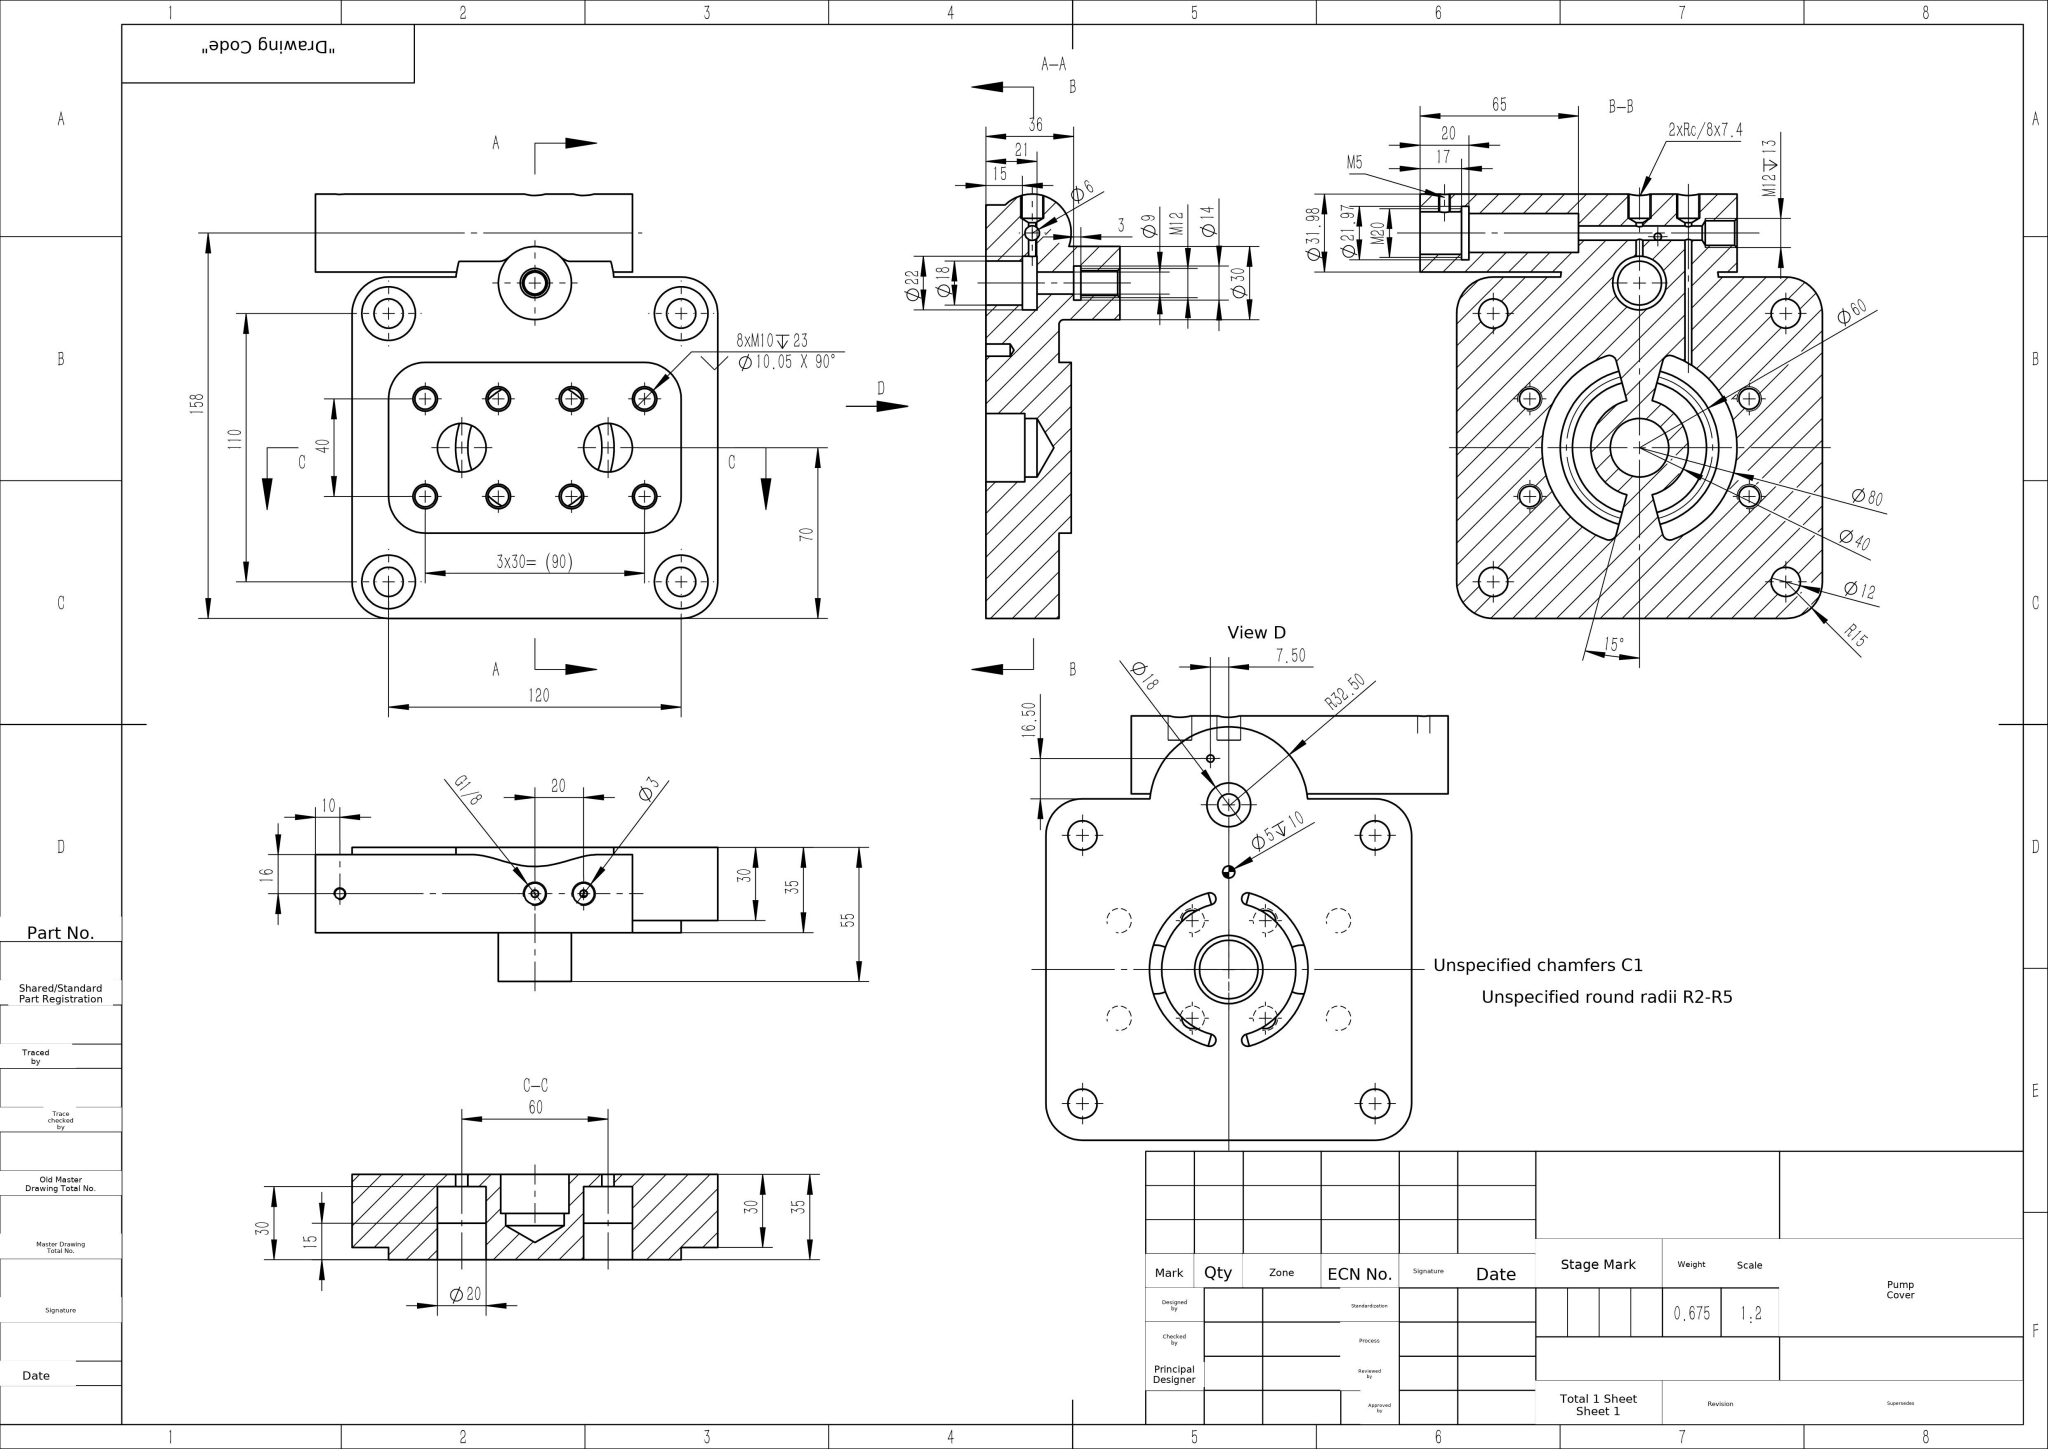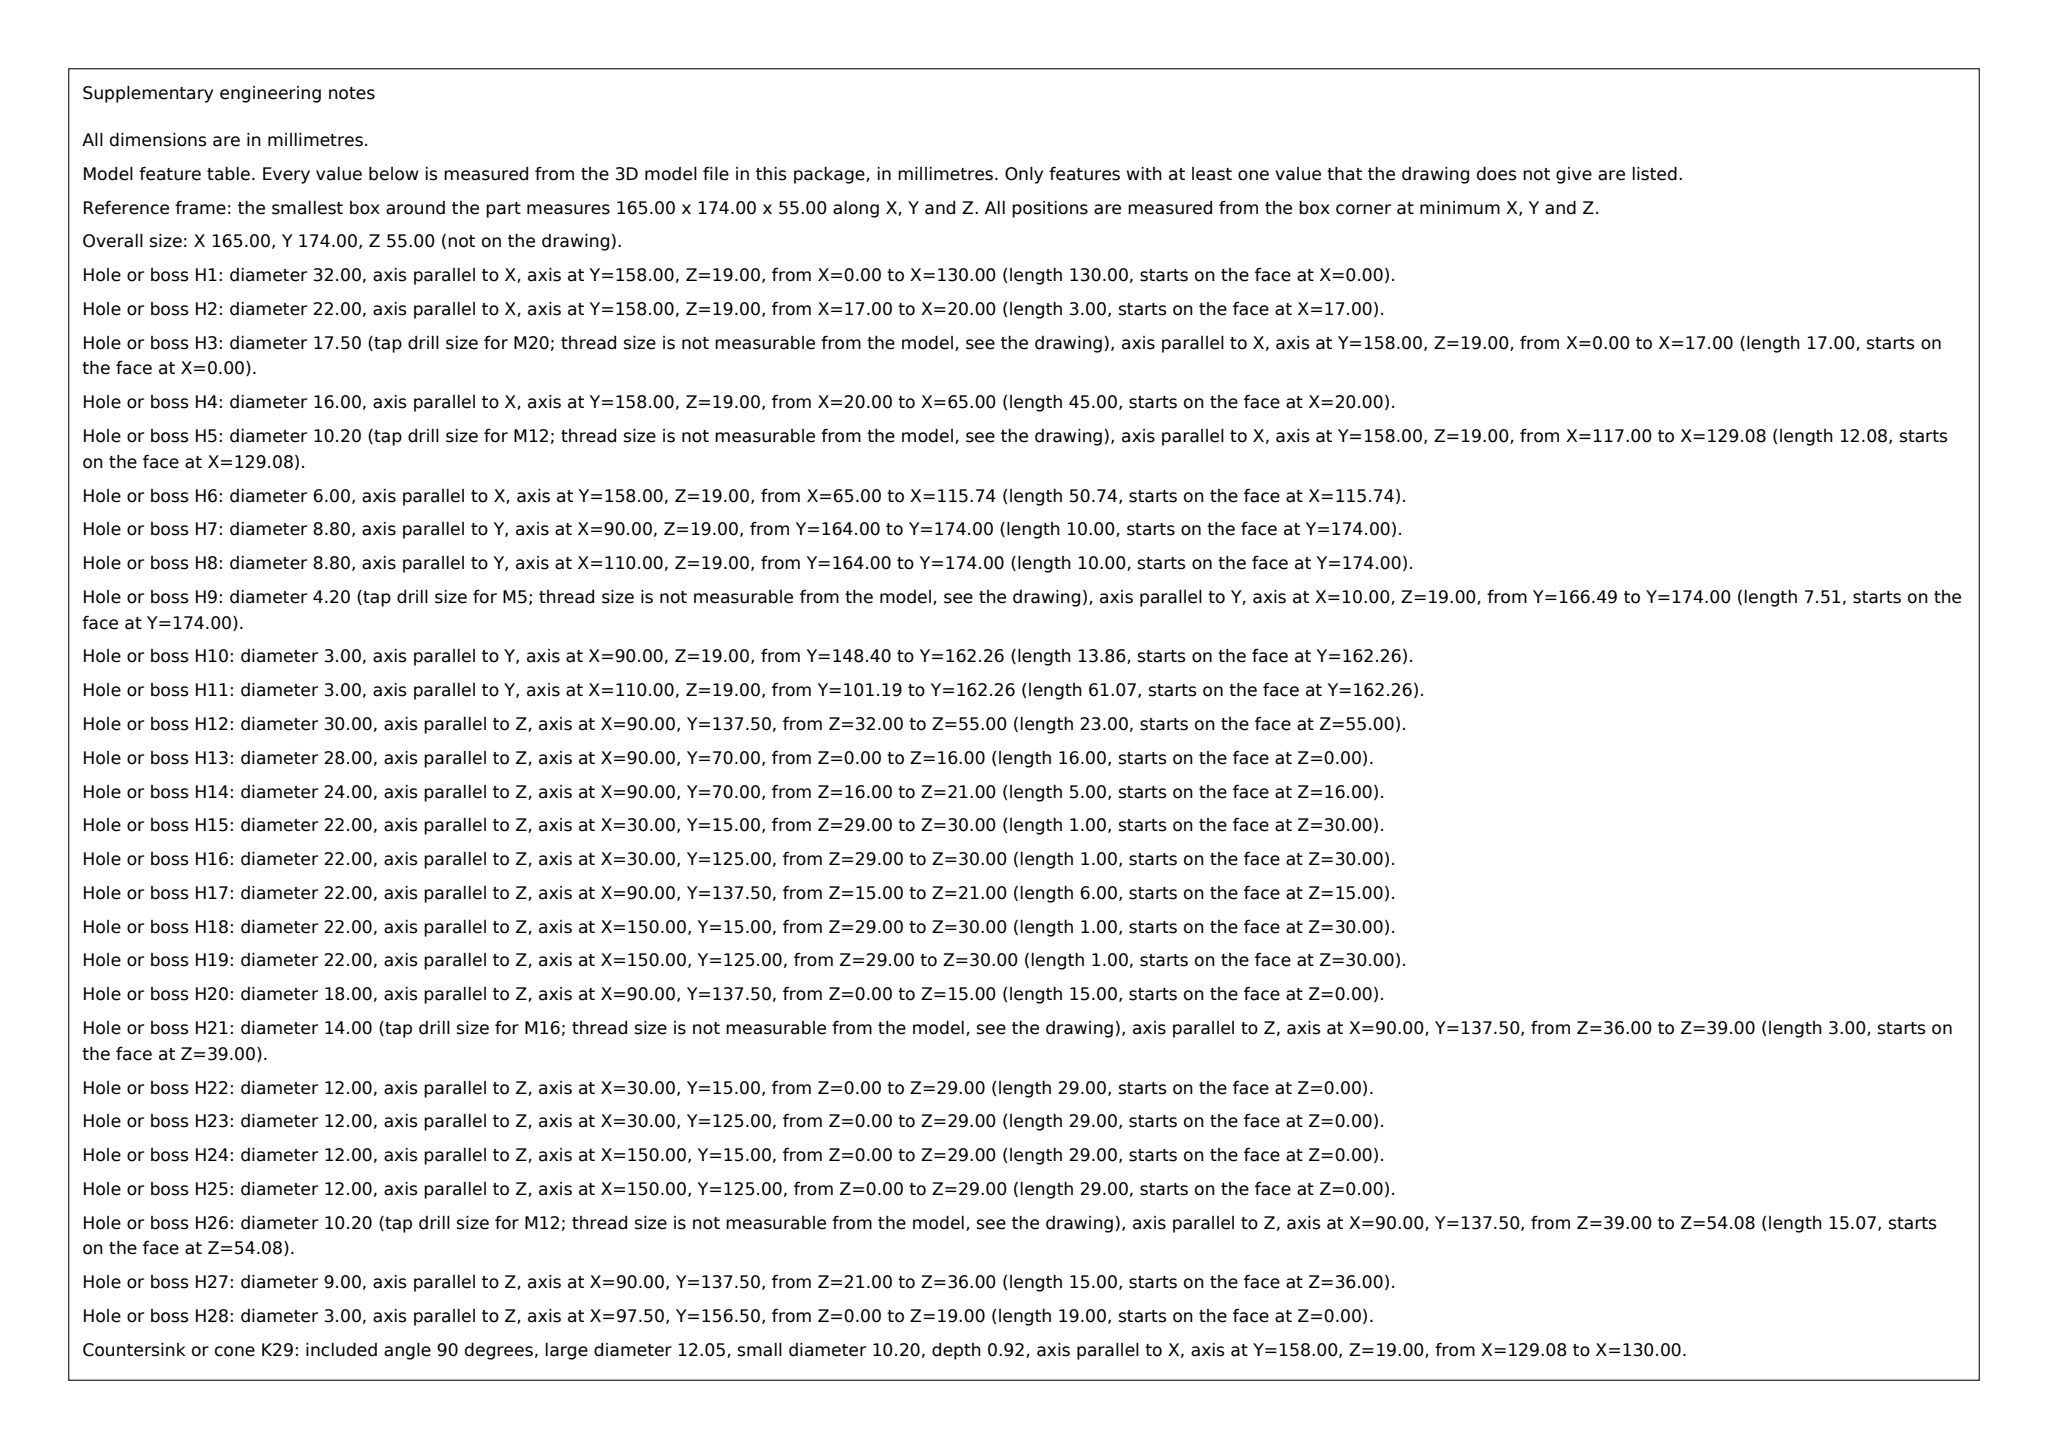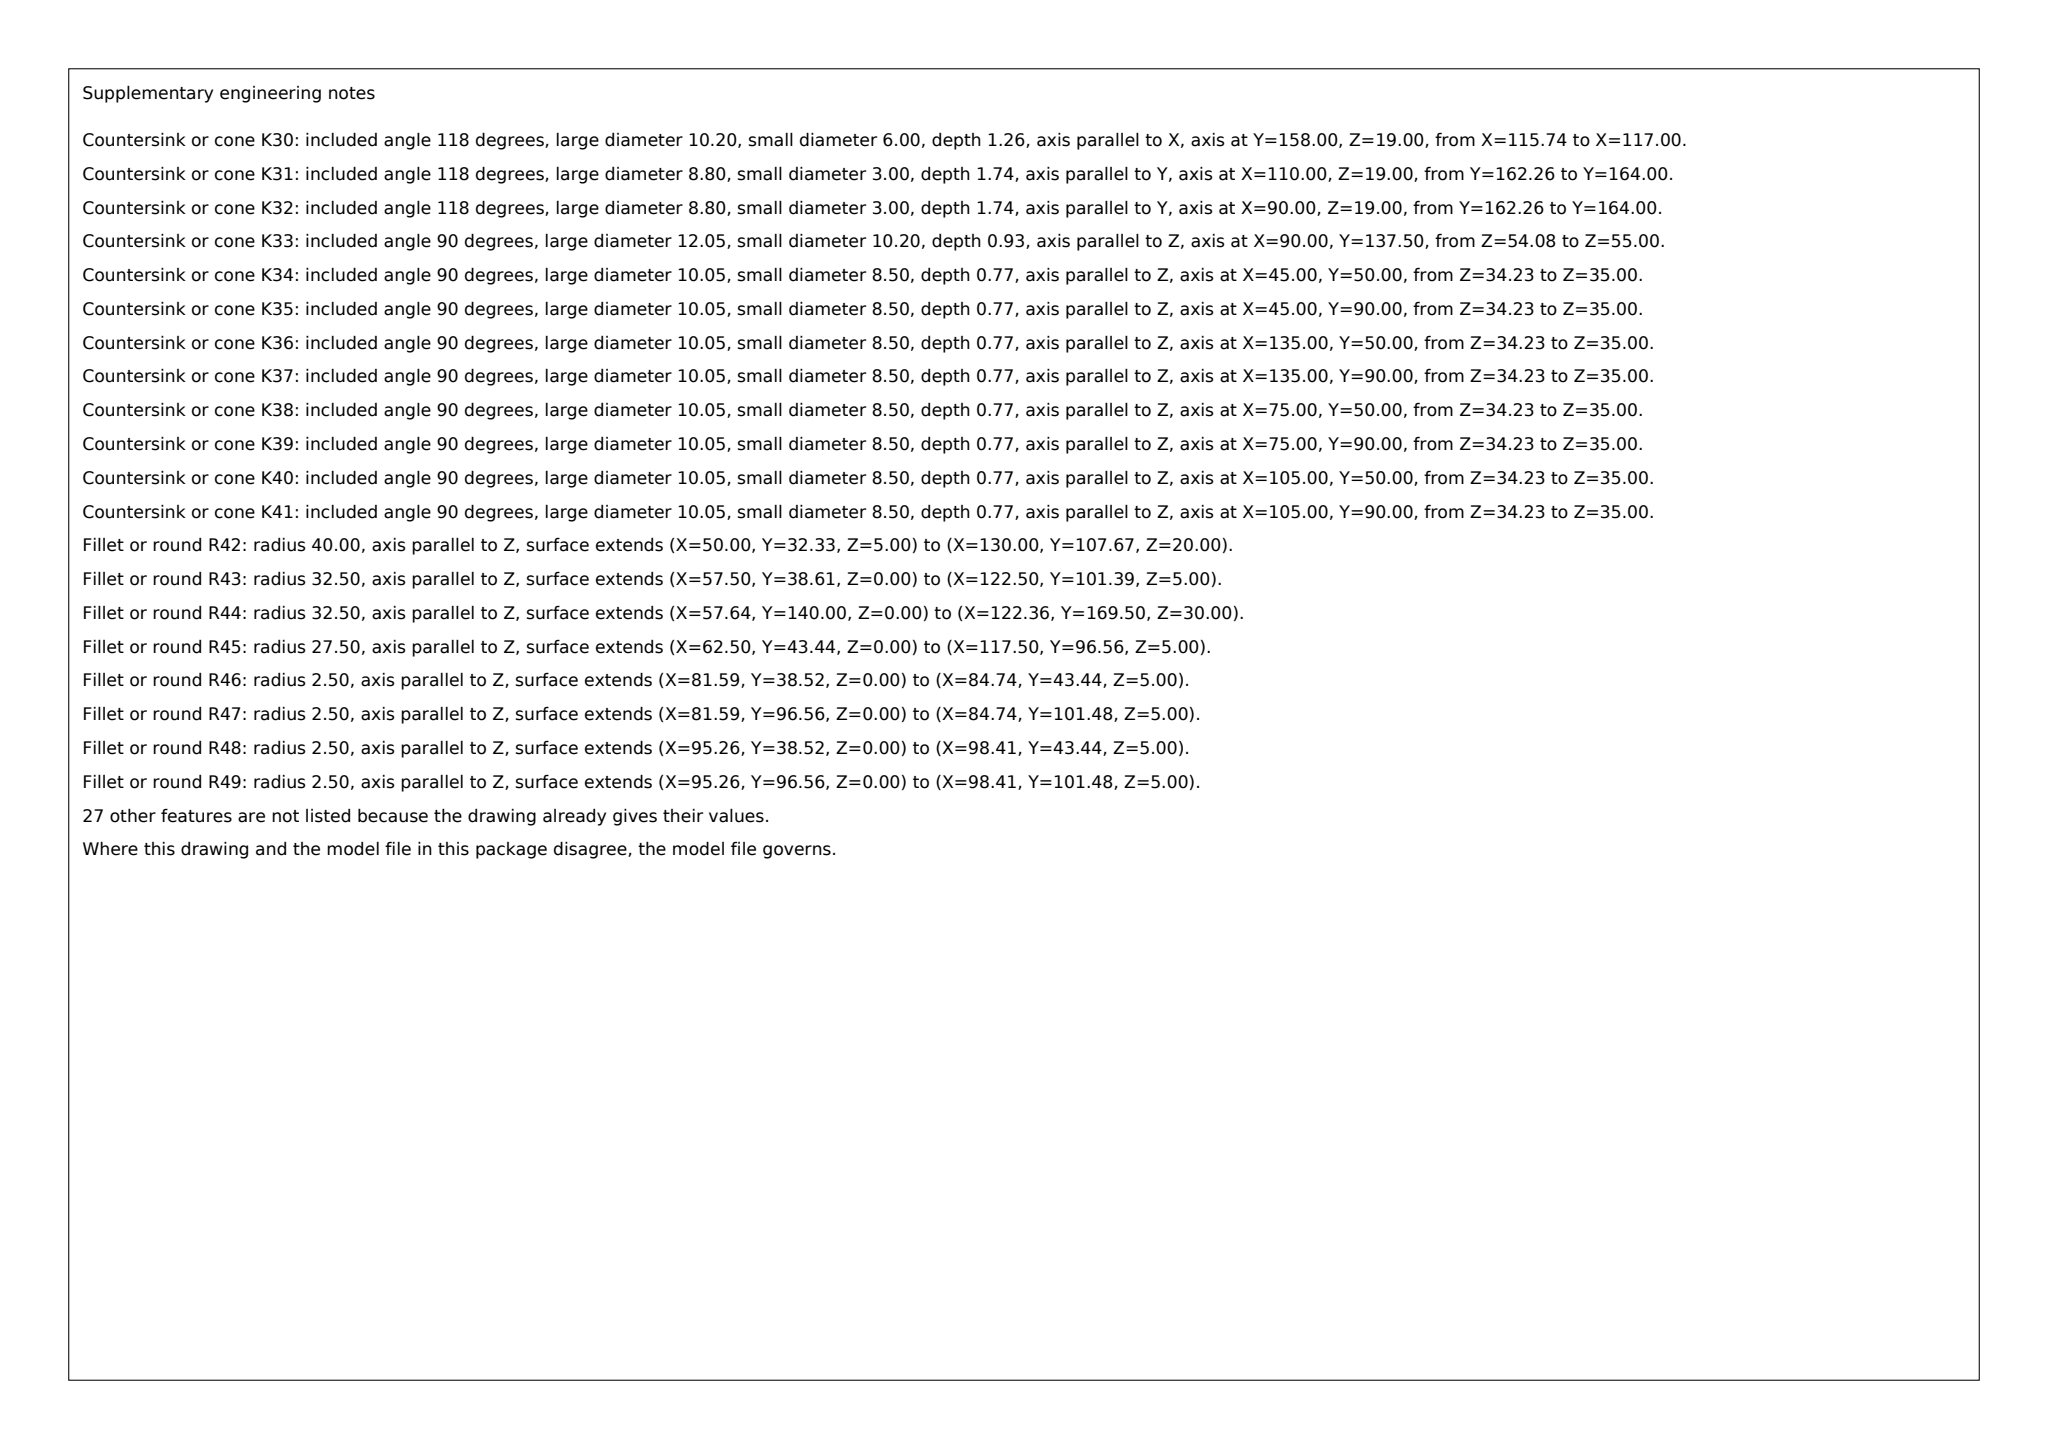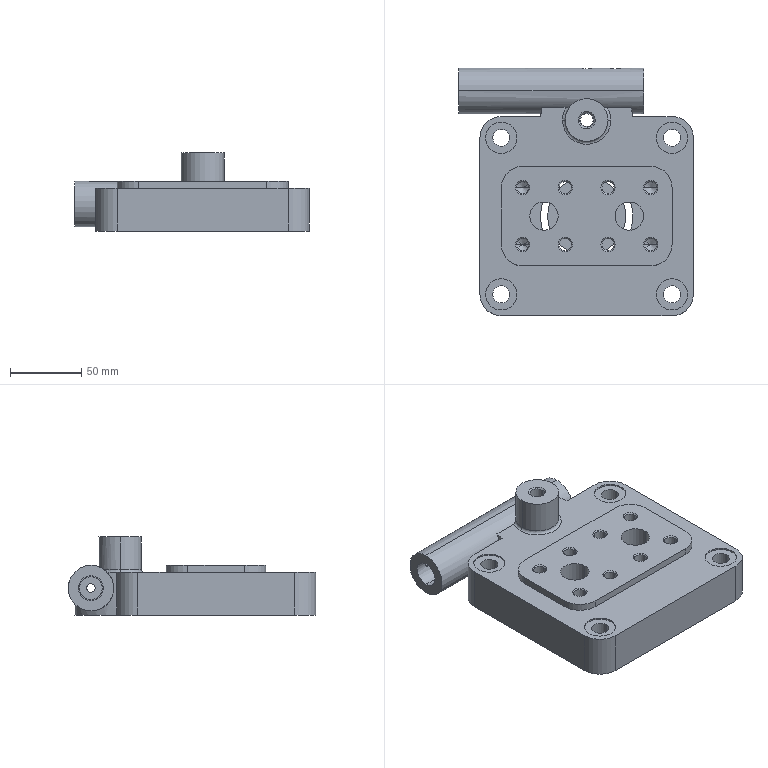Part | SolidWorks | mm | 1 solid | 198 faces | box 165 x 174 x 55 mm | volume 674925 mm3 | cylinder 113 | plane 44 | cone 38 | torus 3 | commonest cylinder face diameters 8.5 x16 22 x12 3 x10 30 x10 5 x8 12 x8 6 x6 10.2 x4